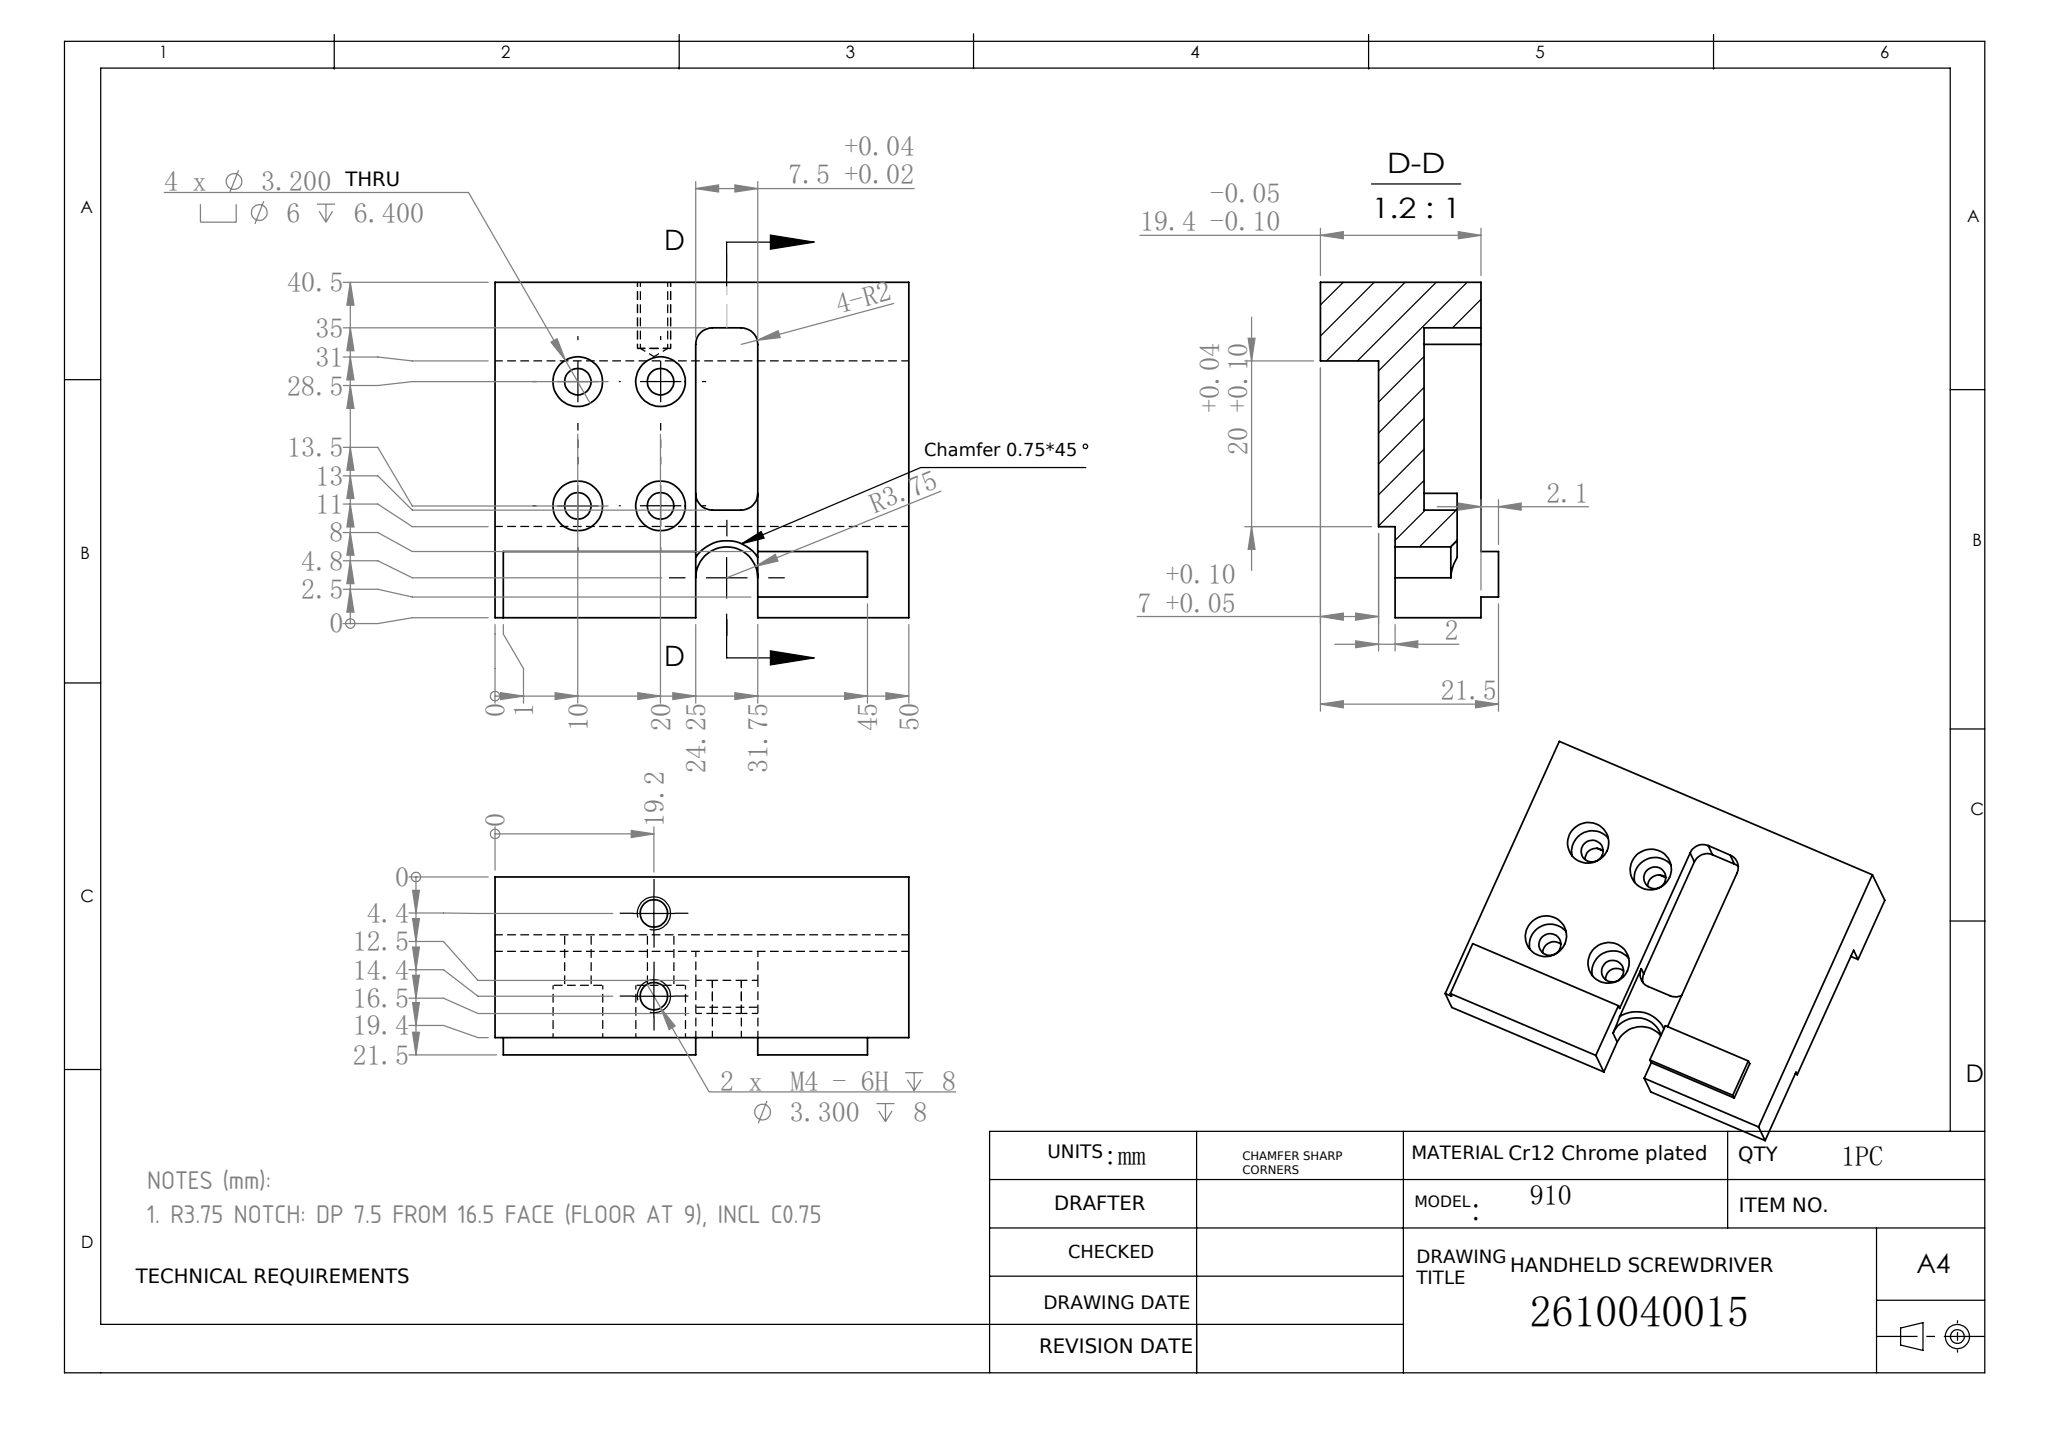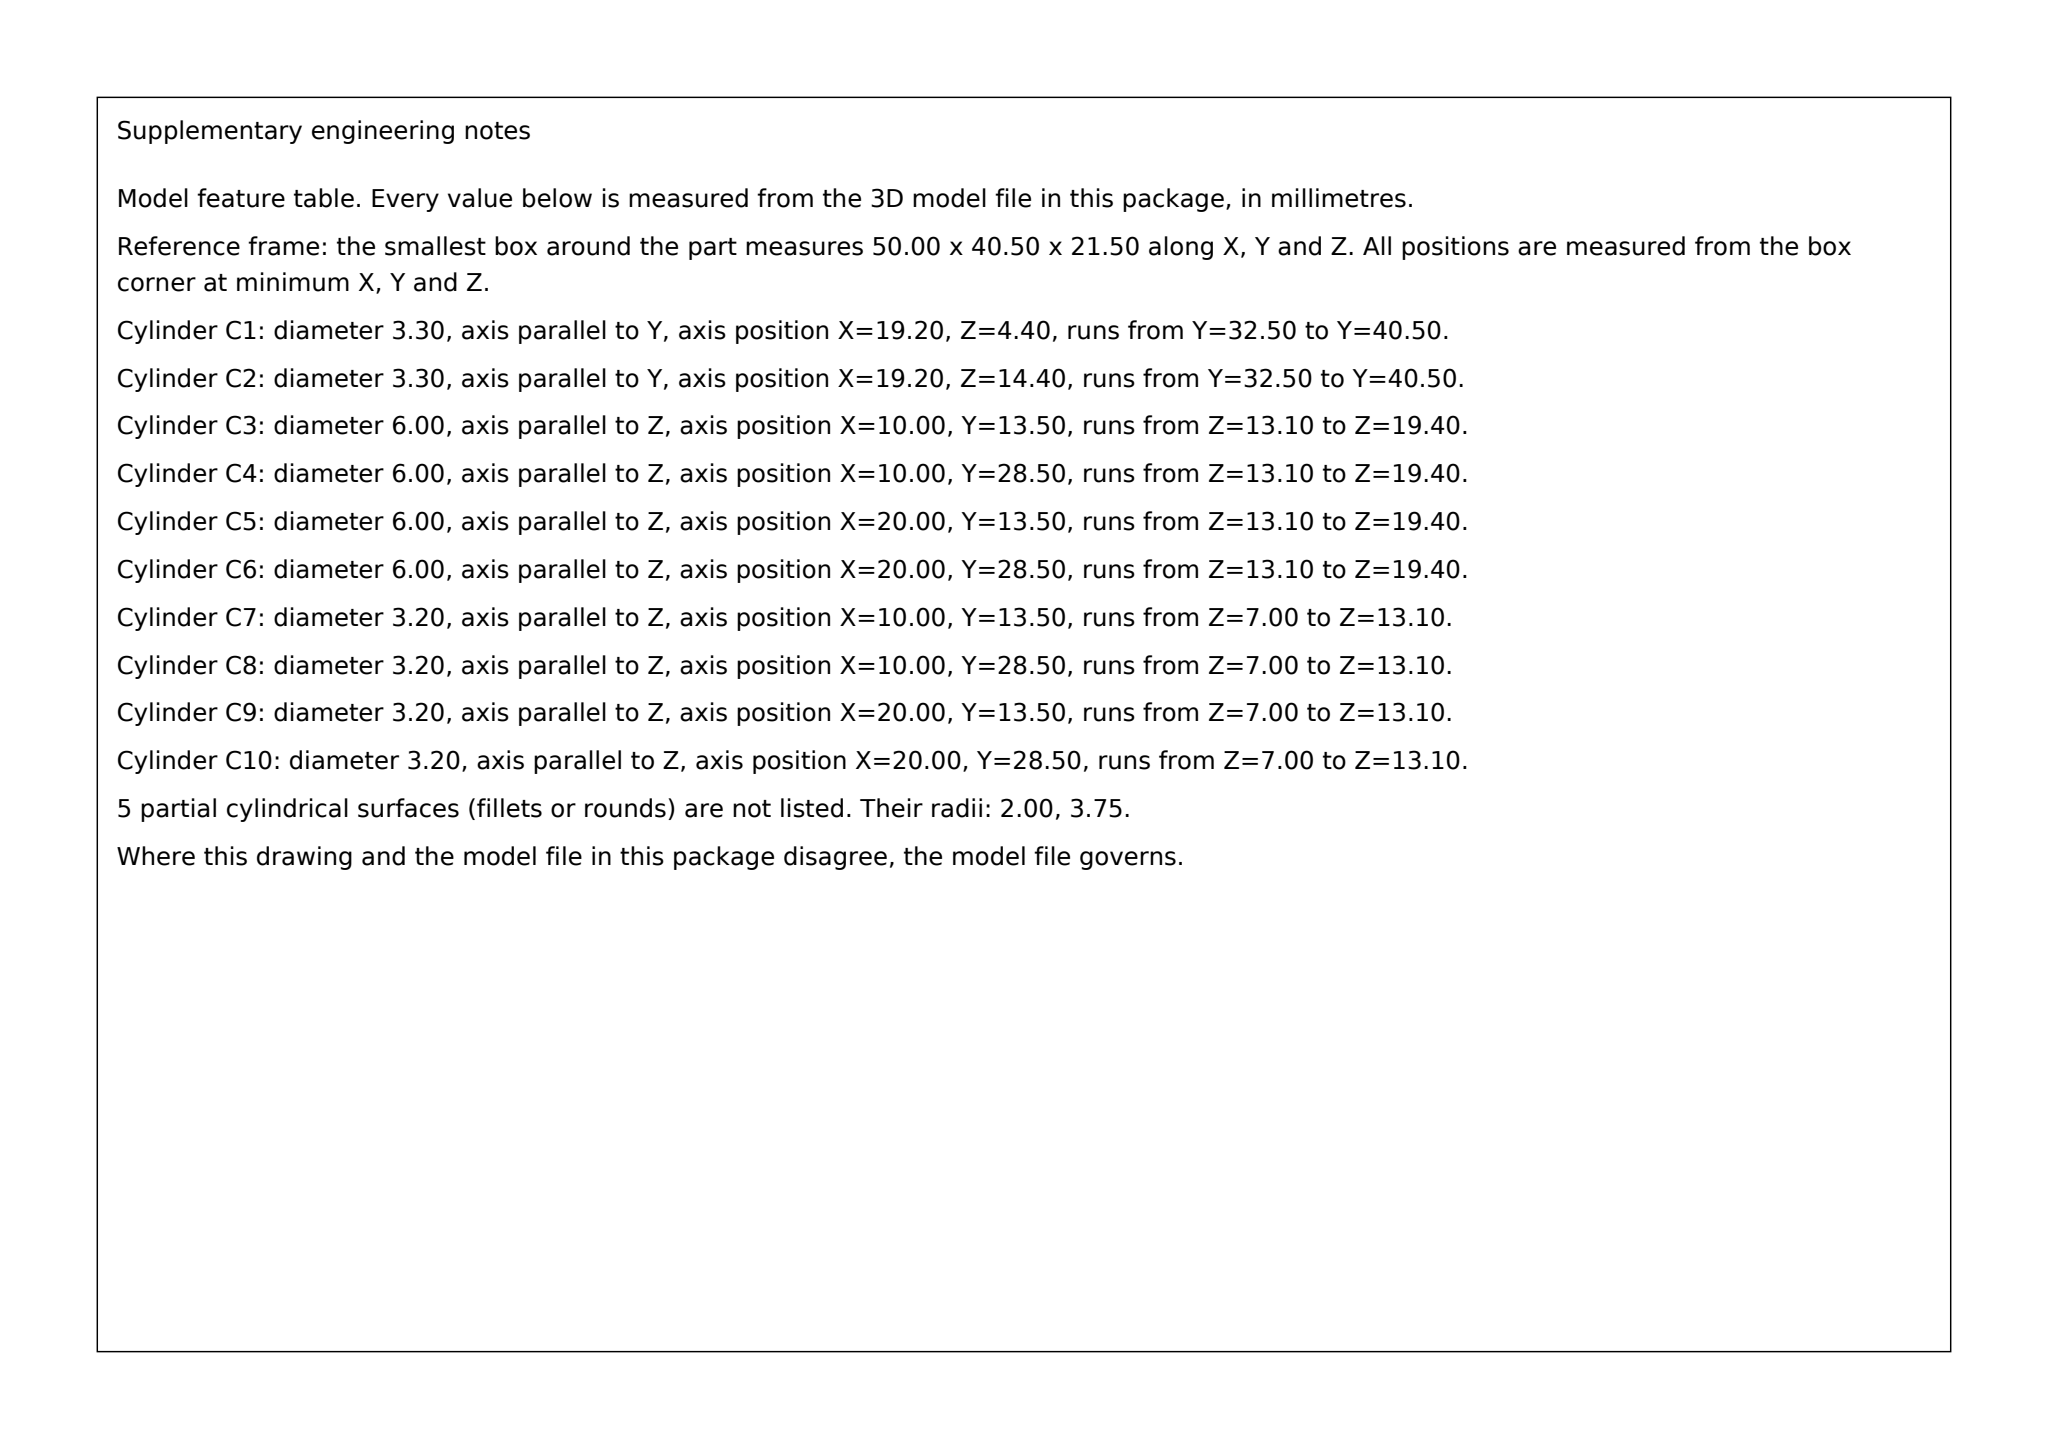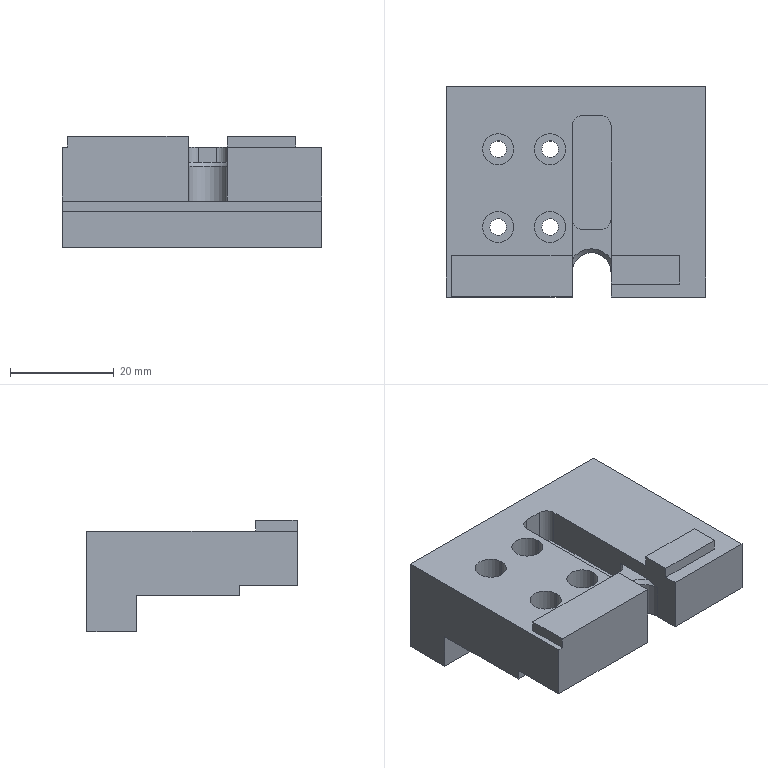Part | SolidWorks | mm | 1 solid | 58 faces | box 50 x 40.5 x 21.5 mm | volume 24986 mm3 | plane 28 | cylinder 25 | cone 5 | commonest cylinder face diameters 3.2 x8 6 x8 3.3 x4 4 x4 7.5 x1
Drawing notes:
R3.75 NOTCH: DP 7.5 FROM 16.5 FACE (FLOOR AT 9), INCL C0.75 | from the solid: cyl dia7.5 axis z at (28,4.8) len 6.75 + 90° cone ref dia 9 (0.75x45 chamfer); z planes 16.5 and 9 -> 7.5 total depth